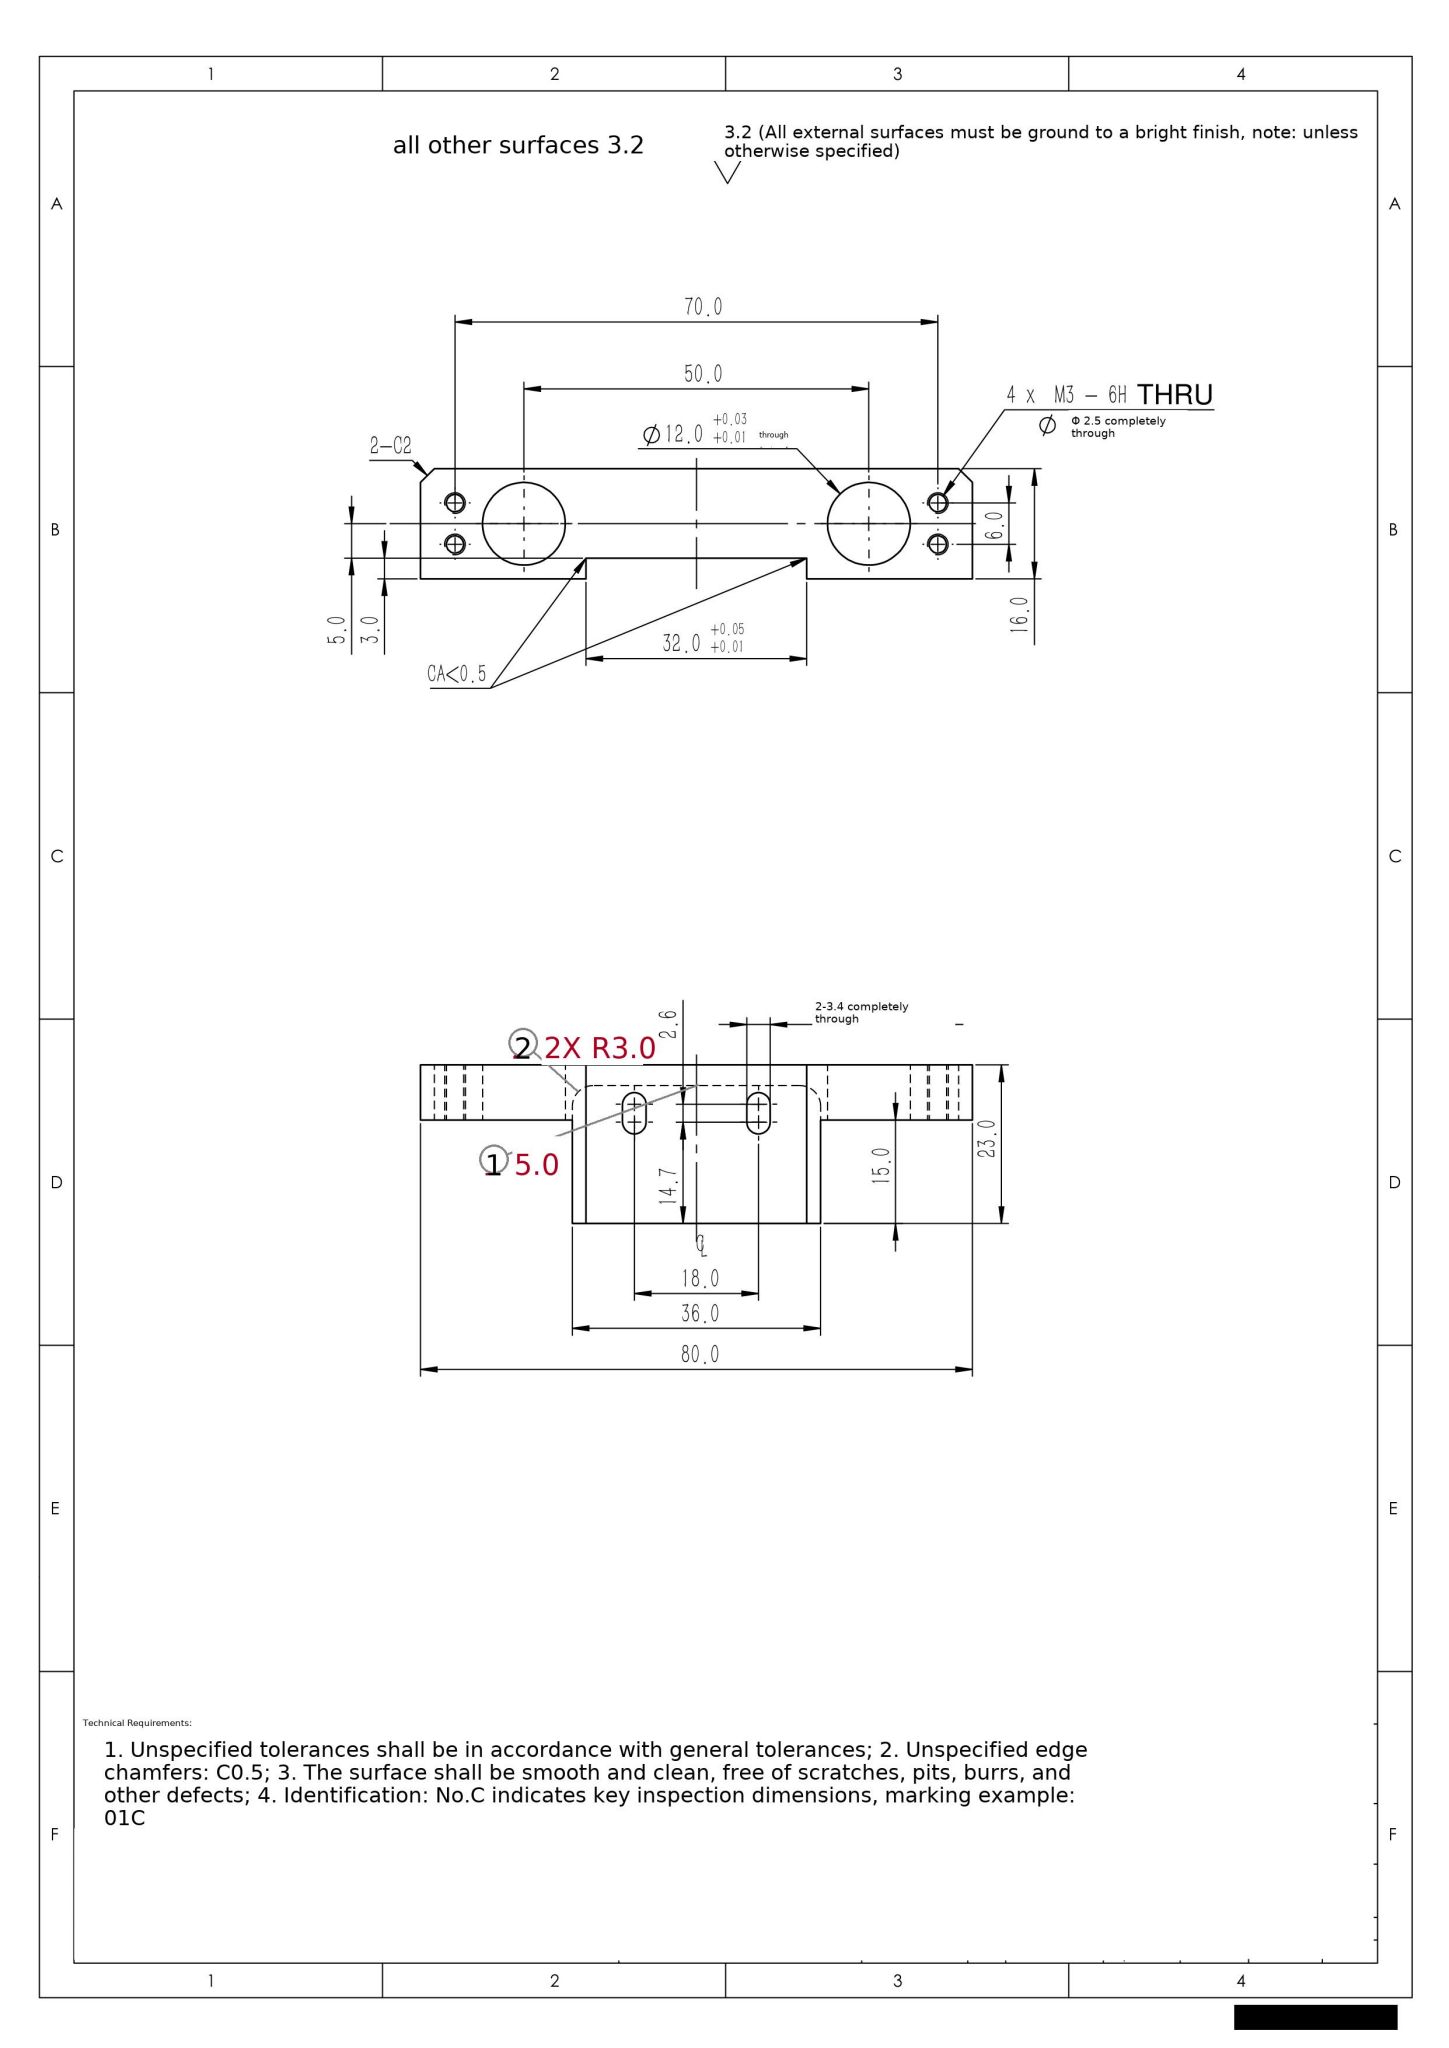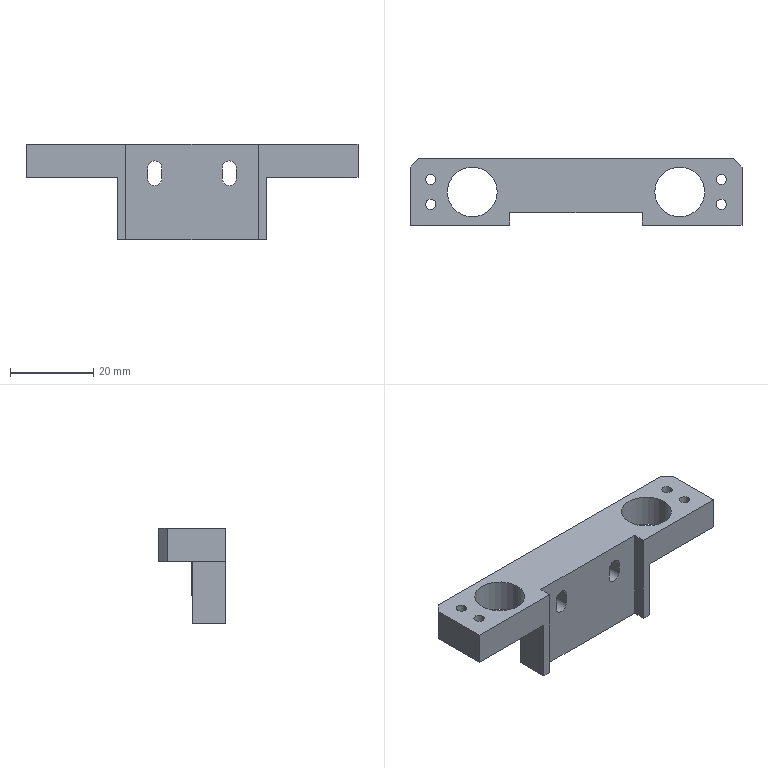Part | SolidWorks | mm | 1 solid | 44 faces | box 80 x 16 x 23 mm | volume 8765 mm3 | plane 24 | cylinder 20 | commonest cylinder face diameters 2.5 x8 3.4 x6 12 x4 6 x2